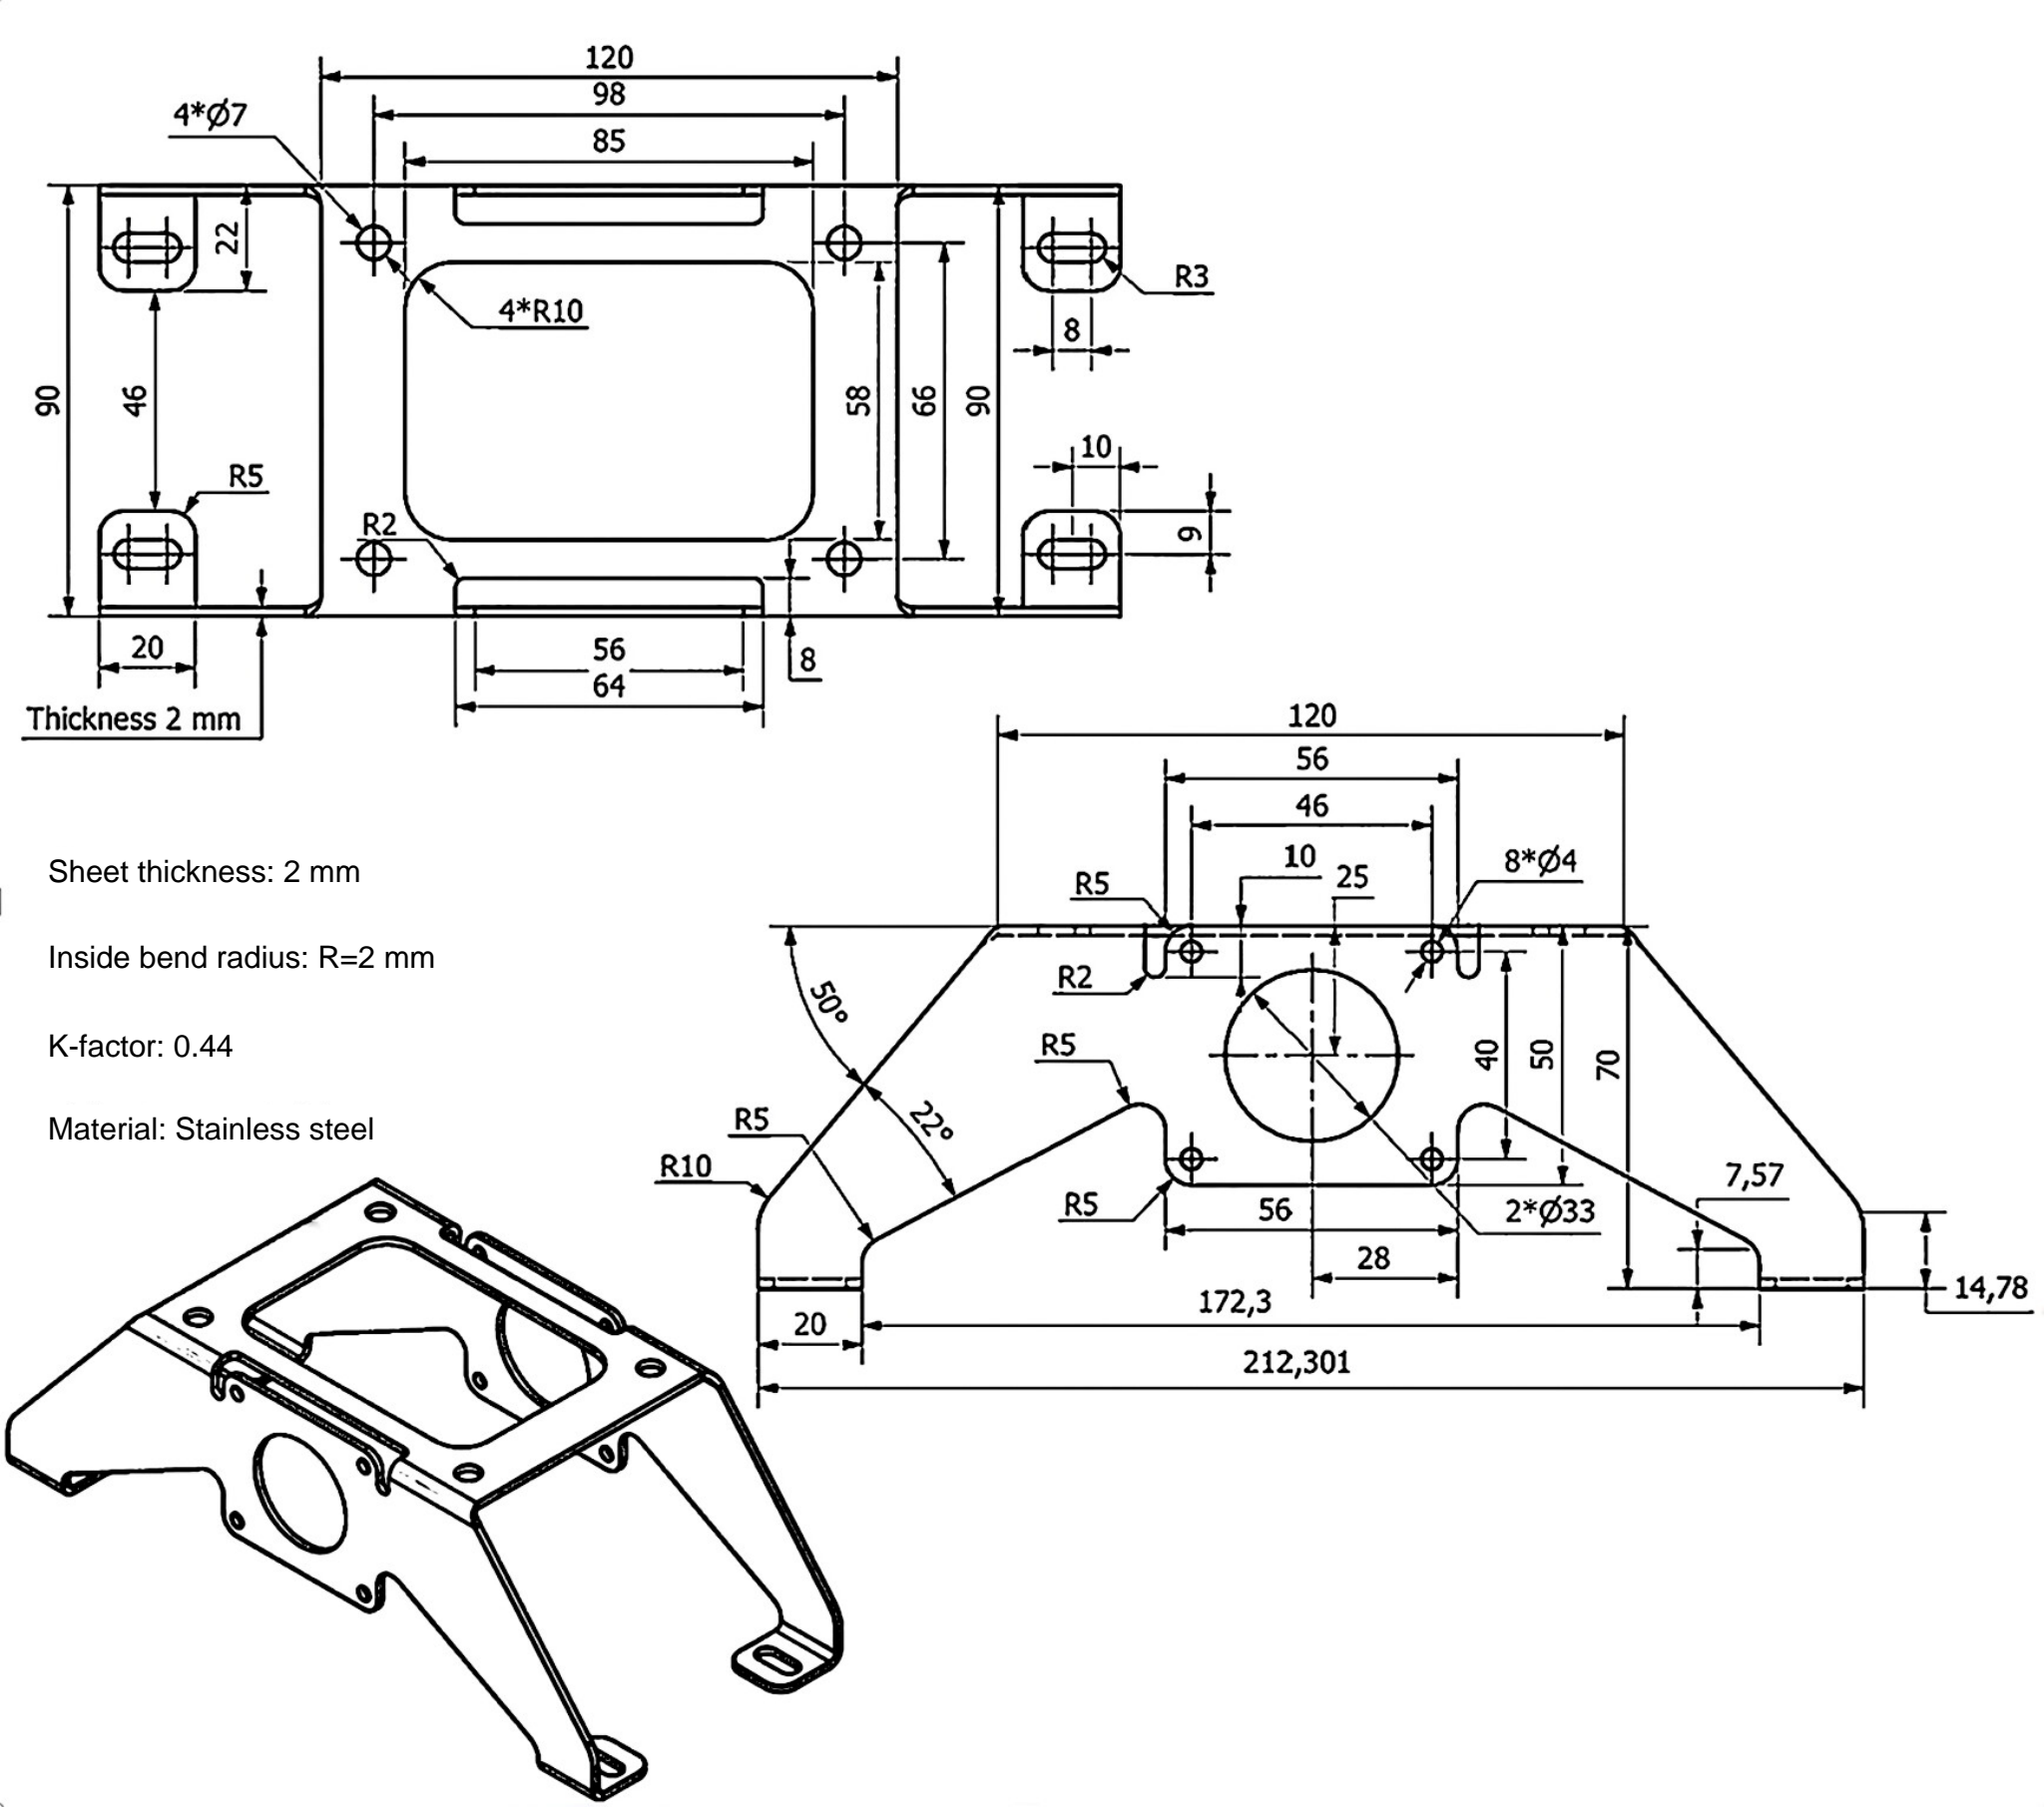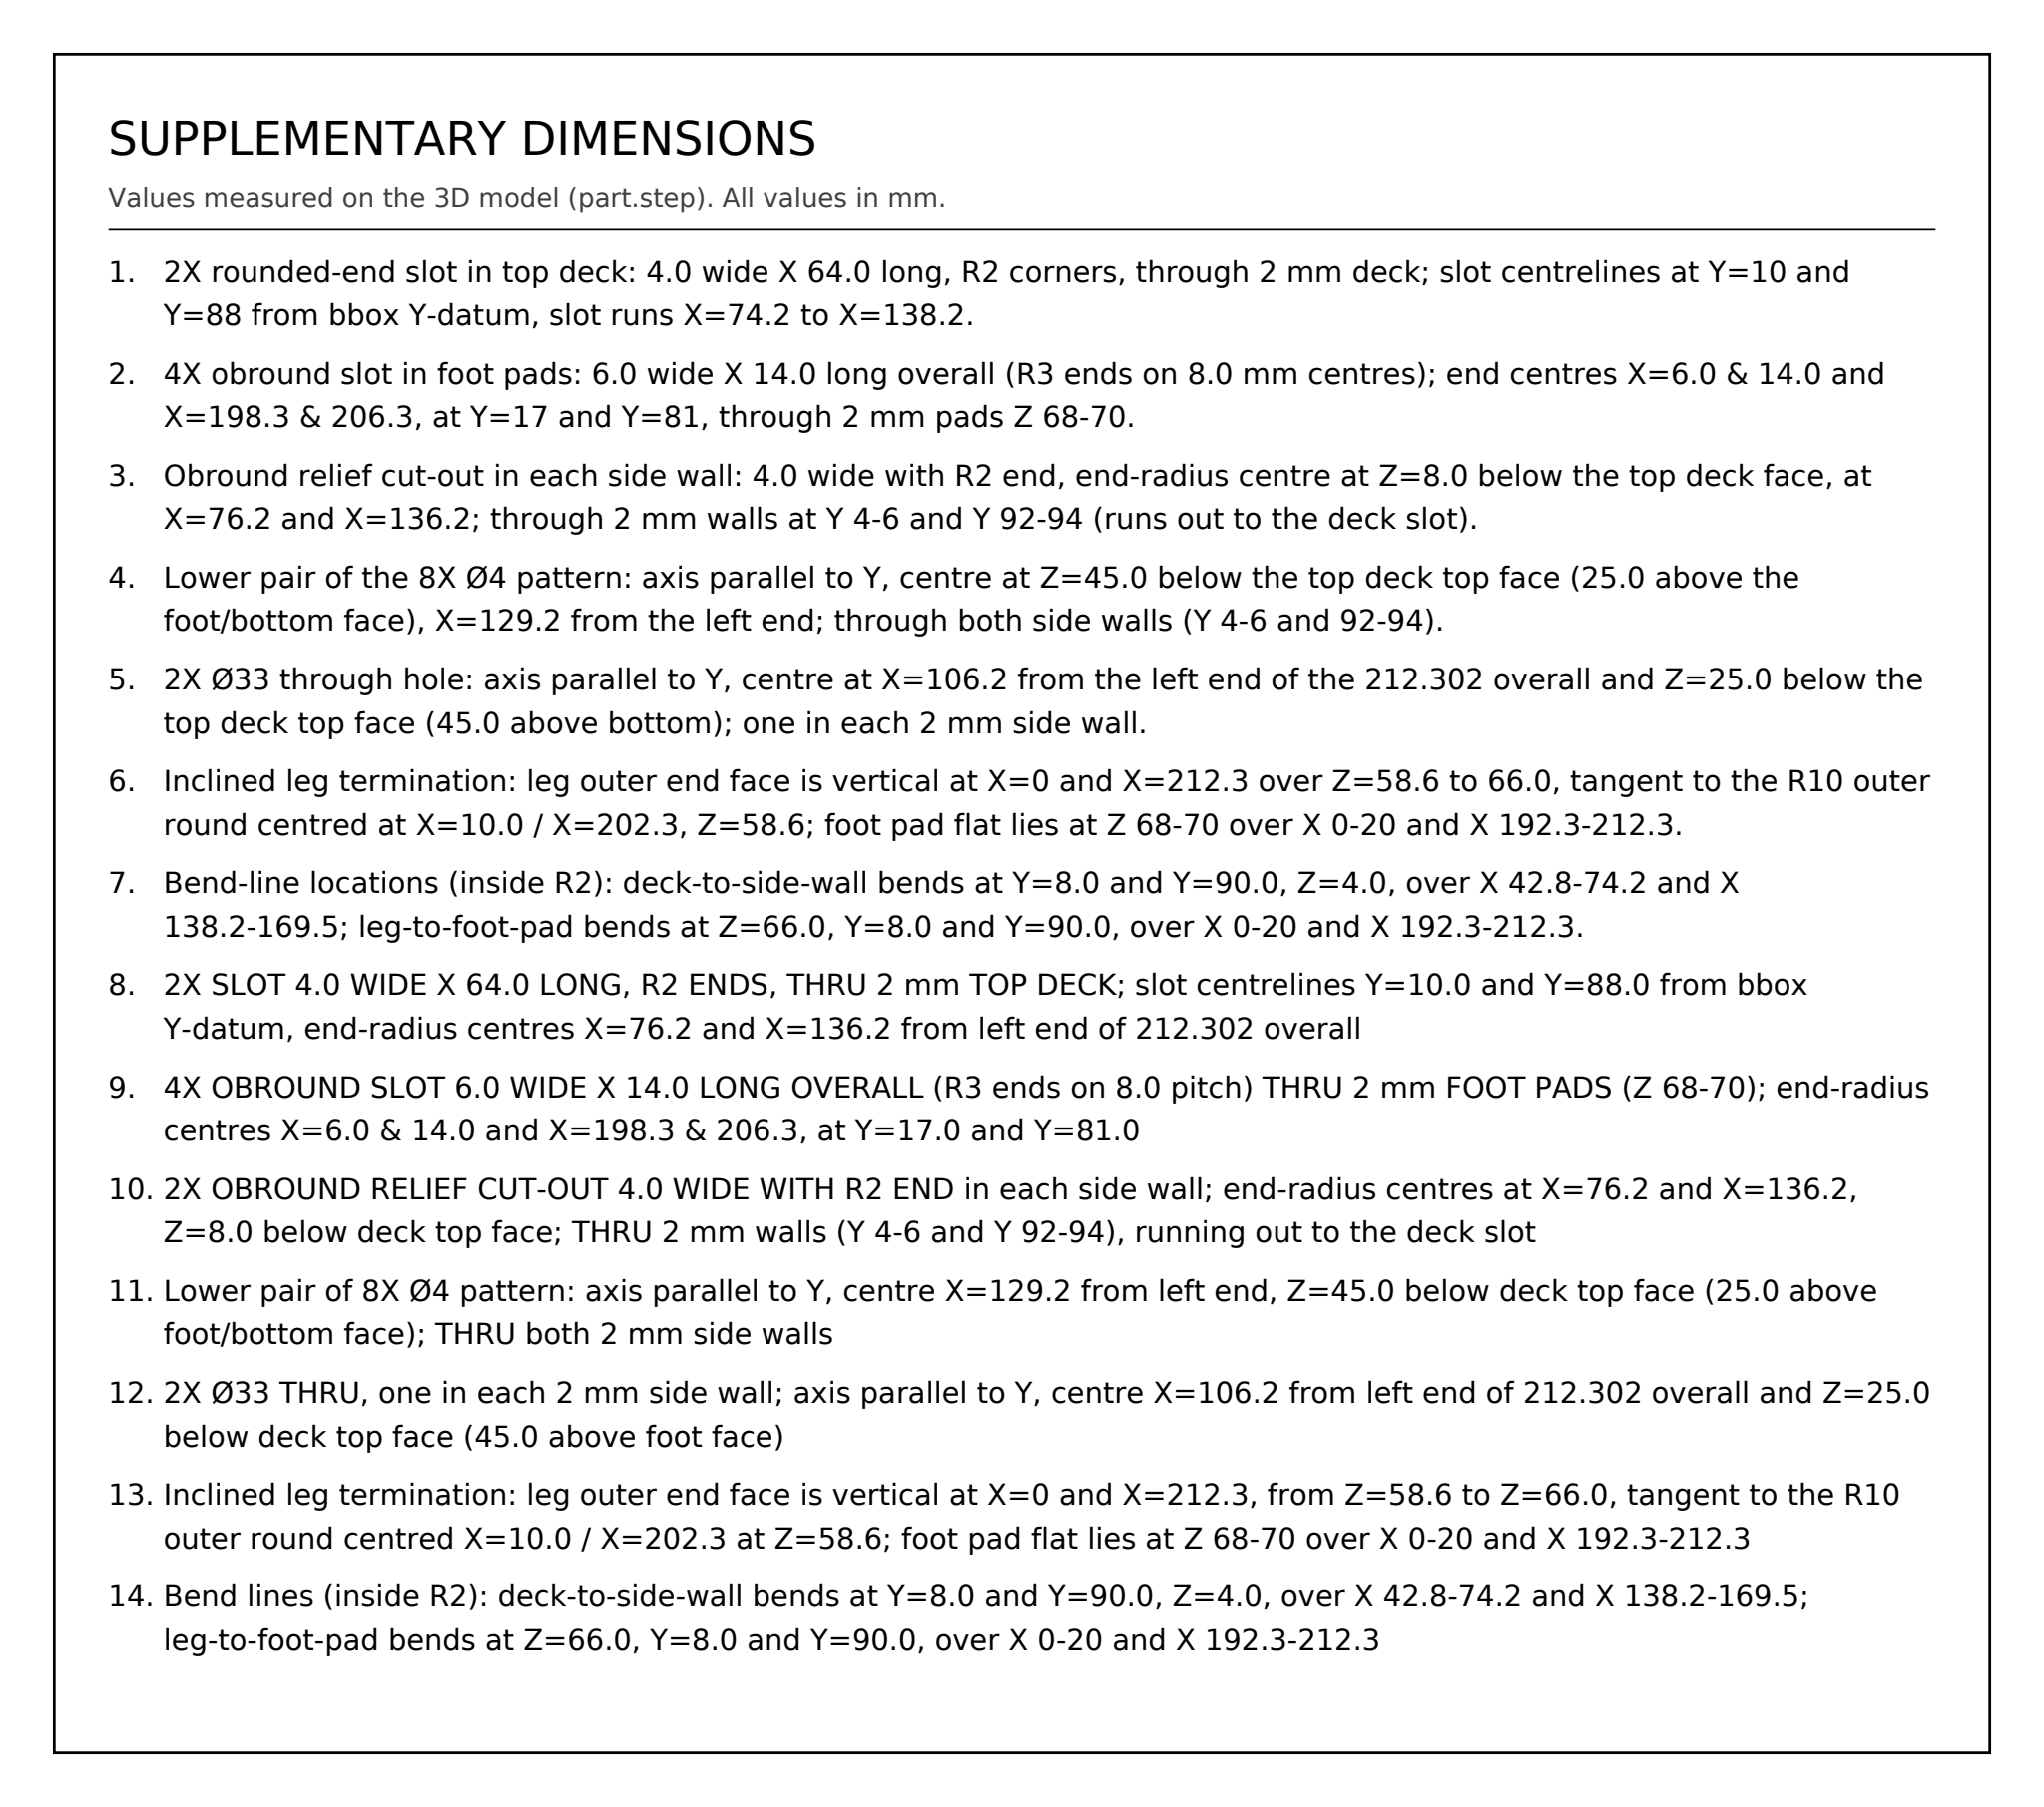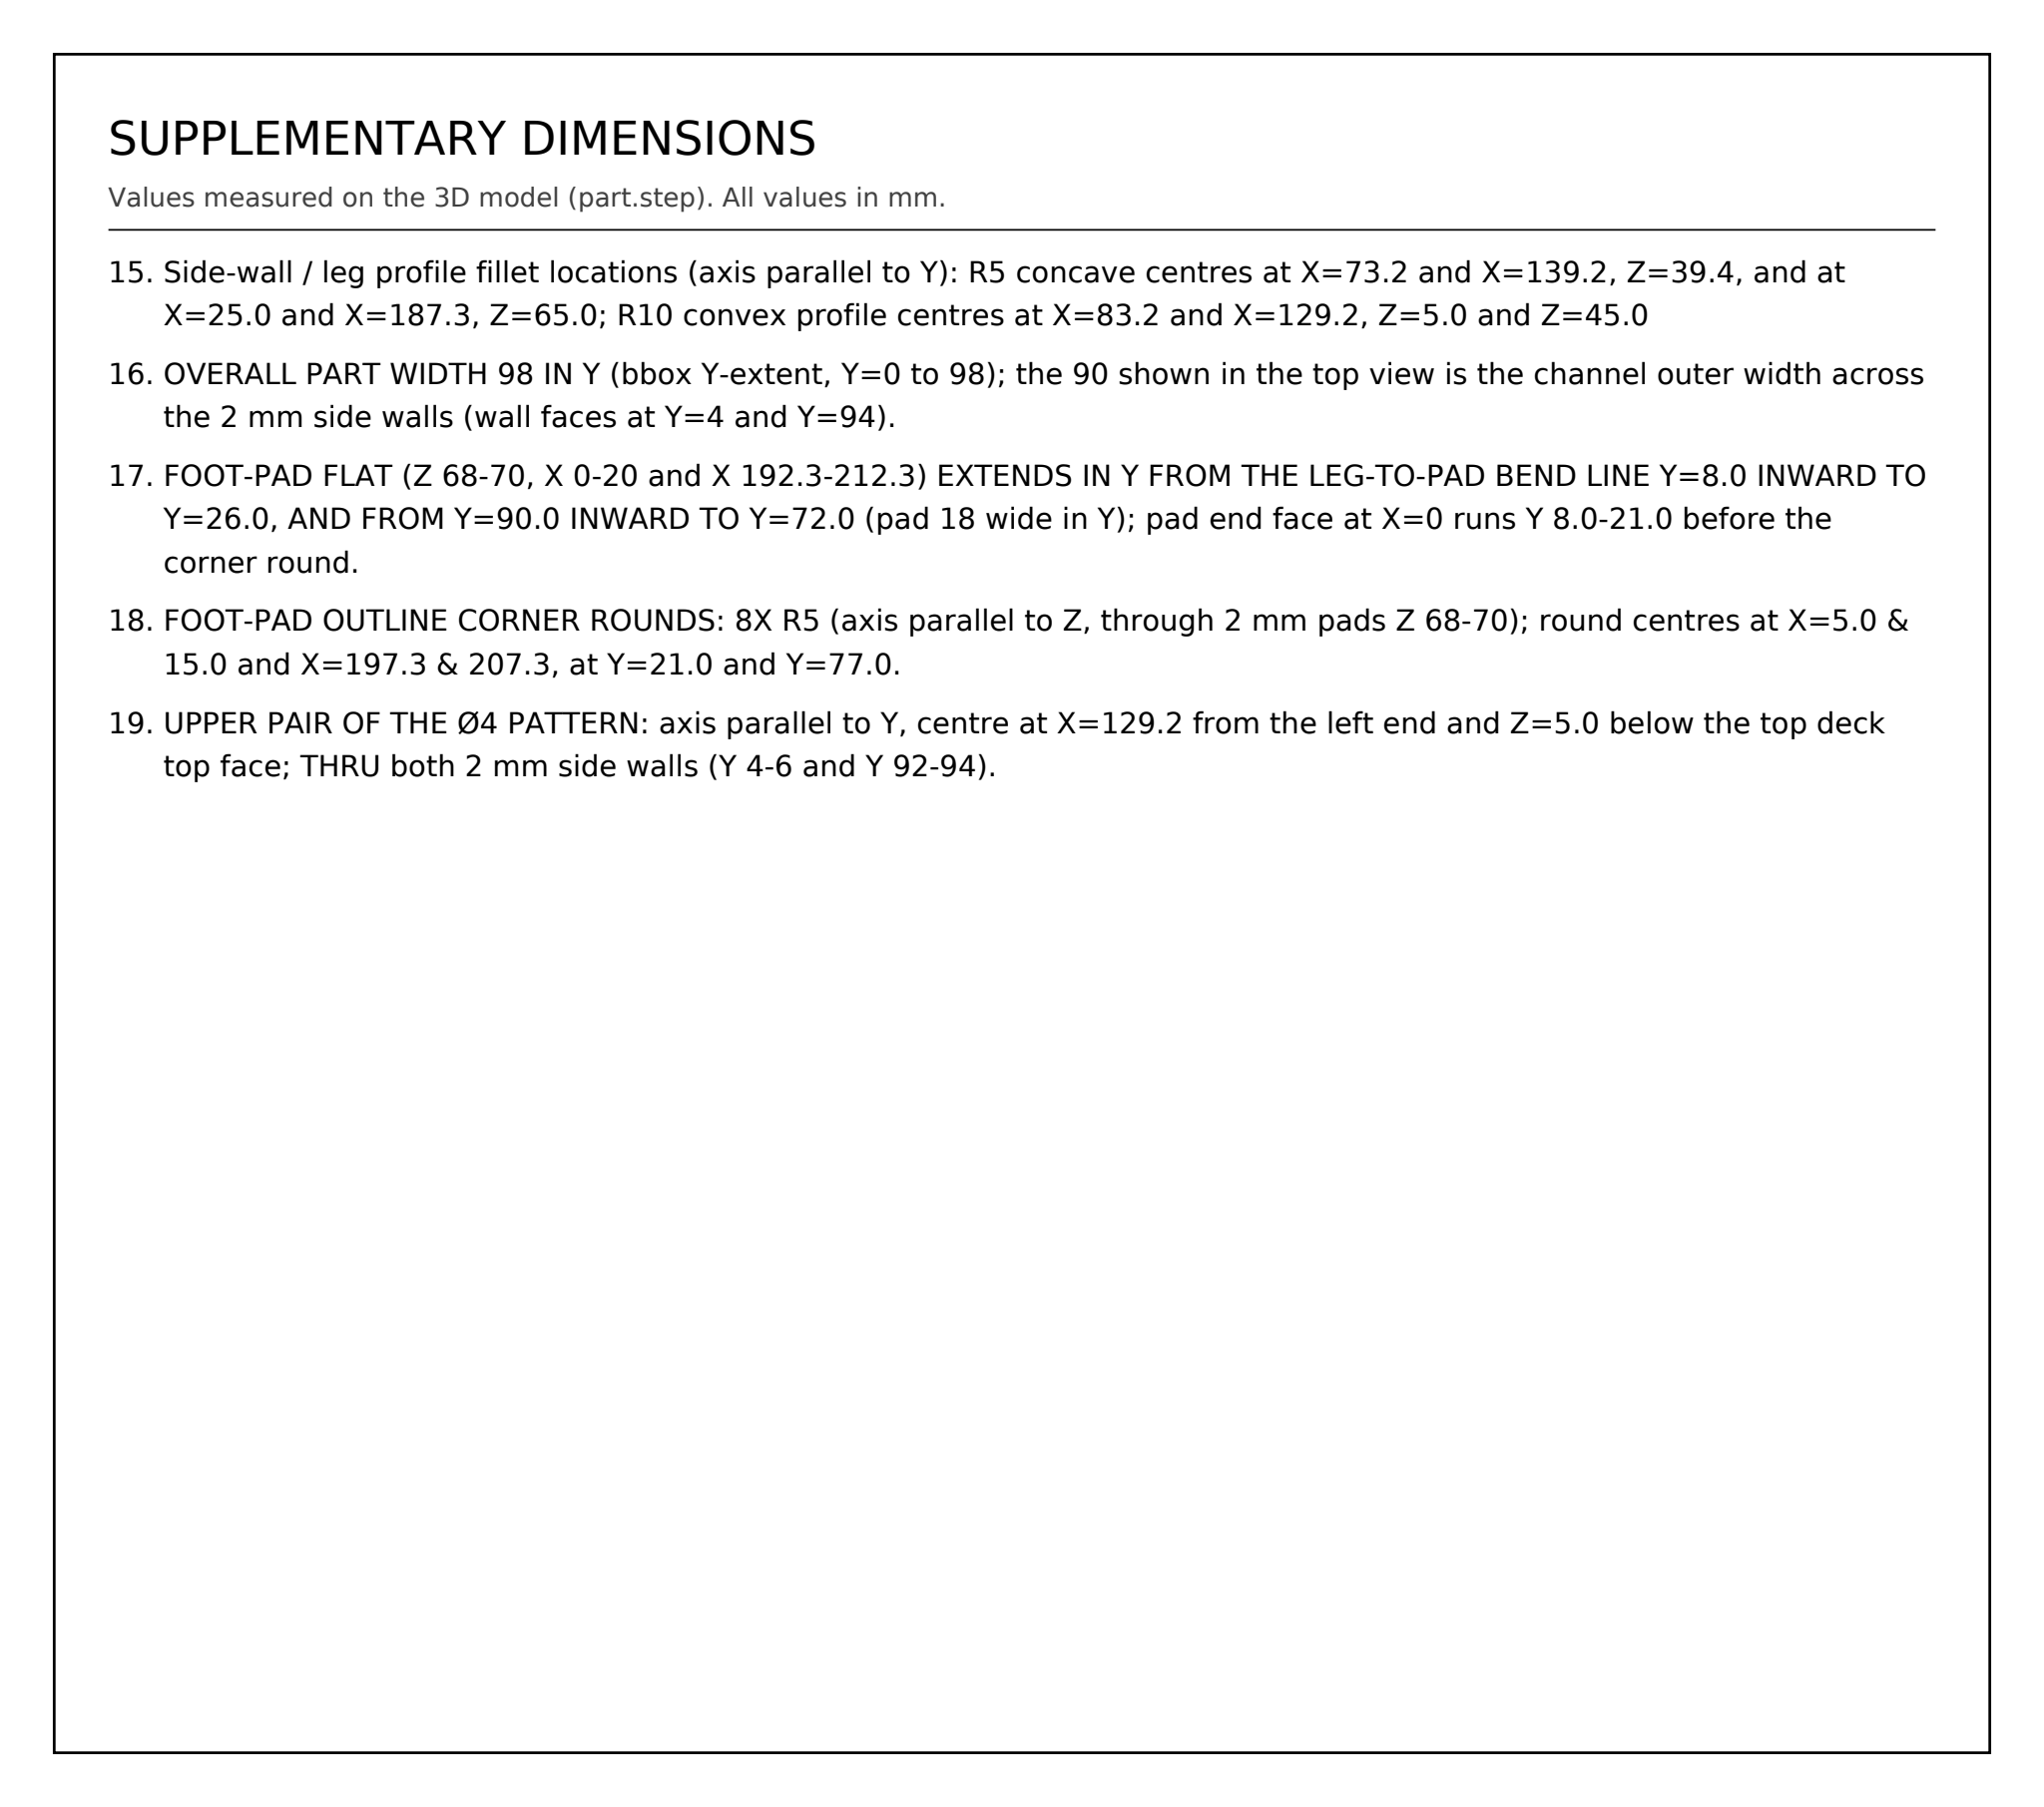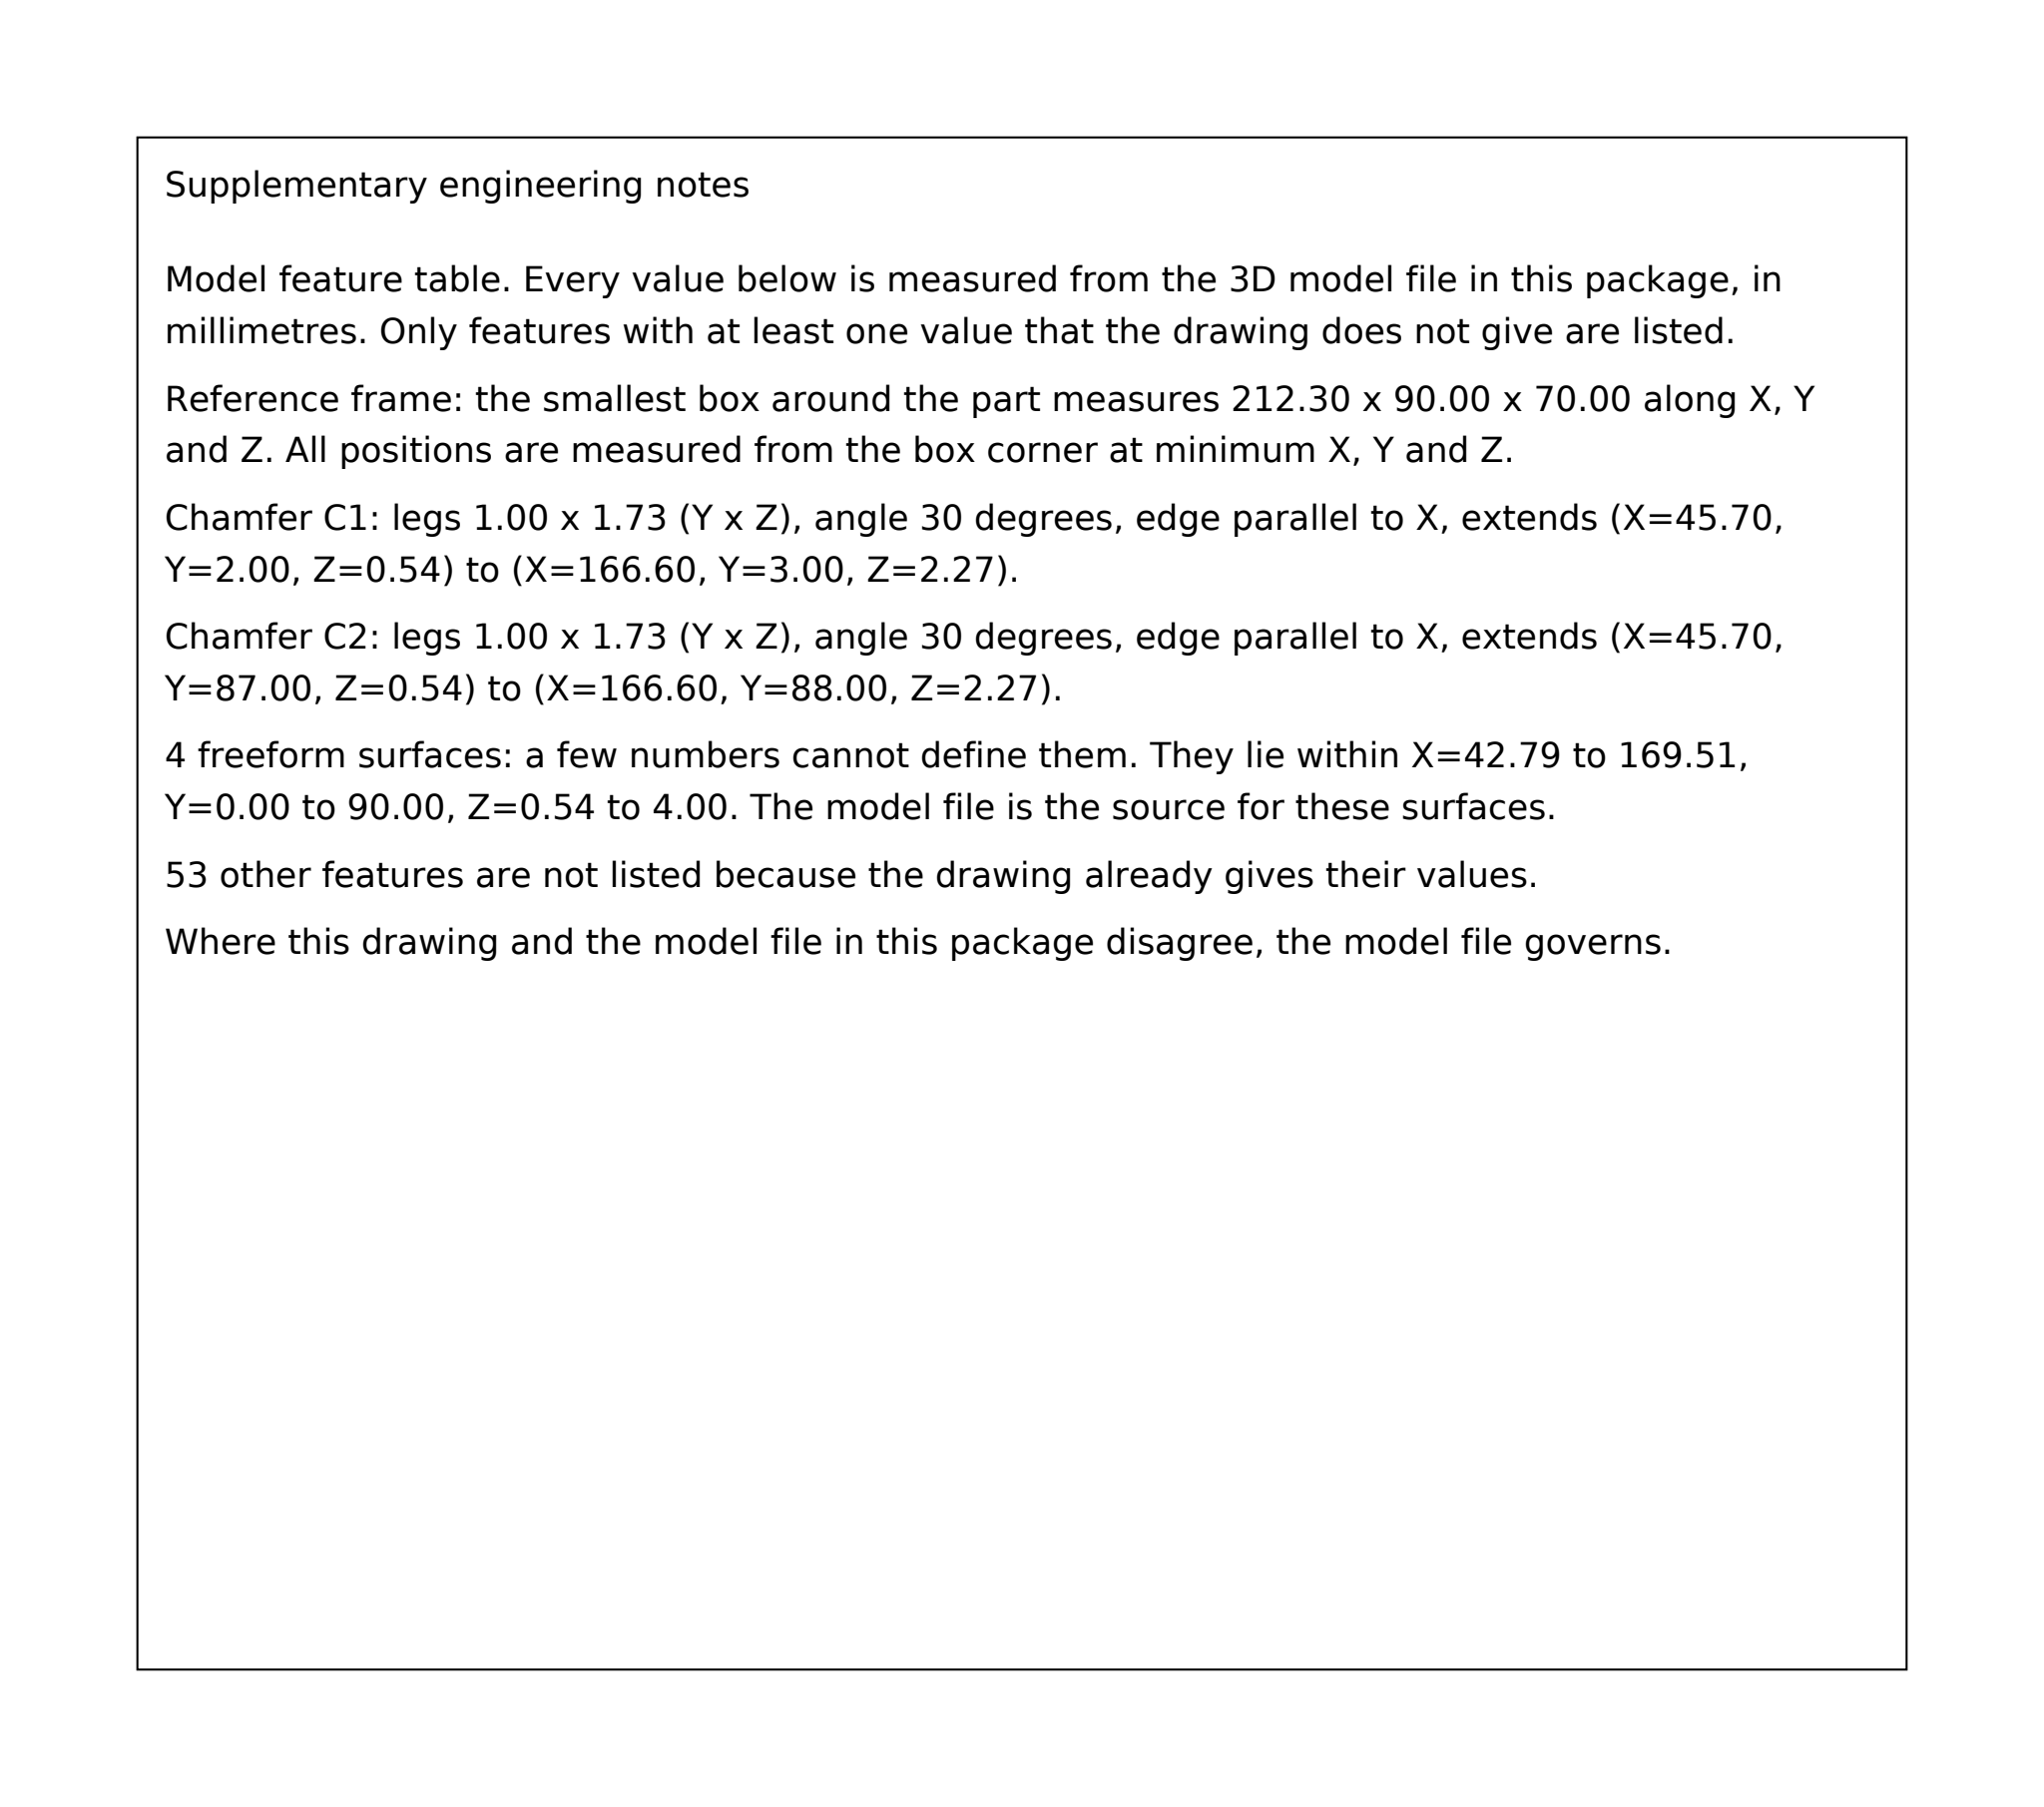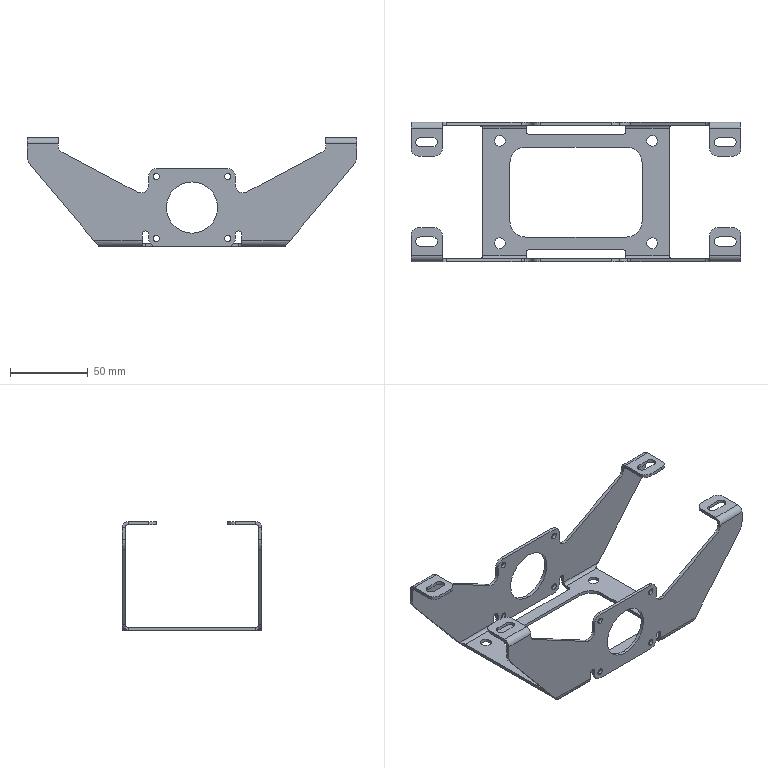Part | SolidWorks | mm | 1 solid | 202 faces | box 212.3 x 90 x 70 mm | volume 41125 mm3 | cylinder 100 | plane 98 | spline 4 | commonest cylinder face diameters 4 x34 10 x26 6 x12 7 x8 20 x8 8 x8 33 x4
Drawing notes:
2X rounded-end slot in top deck: 4.0 wide X 64.0 long, R2 corners, through 2 mm deck; slot centrelines at Y=10 and Y=88 from bbox Y-datum, slot runs X=74.2 to X=138.2. | from the solid: concave arc (R2) dia 4.0, z-axis, at (136.2,10),(76.2,10),(136.2,88),(76.2,88), from z 0.0 to 2.0
4X obround slot in foot pads: 6.0 wide X 14.0 long overall (R3 ends on 8.0 mm centres); end centres X=6.0 & 14.0 and X=198.3 & 206.3, at Y=17 and Y=81, through 2 mm pads Z 68-70. | from the solid: concave arc dia 6.0, z-axis, at (6,17),(14,17),(198.3,17),(206.3,17),(6,81),(14,81),(198.3,81),(206.3,81), from z 68.0 to 70.0
Obround relief cut-out in each side wall: 4.0 wide with R2 end, end-radius centre at Z=8.0 below the top deck face, at X=76.2 and X=136.2; through 2 mm walls at Y 4-6 and Y 92-94 (runs out to the deck slot). | from the solid: concave arc dia 4.0, y-axis, at (136.2, z=8.0) and (76.2, z=8.0), 180 deg, y 4.0-6.0 and 92.0-94.0
Lower pair of the 8X Ø4 pattern: axis parallel to Y, centre at Z=45.0 below the top deck top face (25.0 above the foot/bottom face), X=129.2 from the left end; through both side walls (Y 4-6 and 92-94). | from the solid: hole/bore dia 4.0, y-axis, at (129.2, z=45.0), from y 4.0 to 6.0 and y 92.0 to 94.0
2X Ø33 through hole: axis parallel to Y, centre at X=106.2 from the left end of the 212.302 overall and Z=25.0 below the top deck top face (45.0 above bottom); one in each 2 mm side wall. | from the solid: hole/bore dia 33.0, y-axis, at (106.2, z=25.0), from y 4.0 to 6.0 and y 92.0 to 94.0
Inclined leg termination: leg outer end face is vertical at X=0 and X=212.3 over Z=58.6 to 66.0, tangent to the R10 outer round centred at X=10.0 / X=202.3, Z=58.6; foot pad flat lies at Z 68-70 over X 0-20 and X 192.3-212.3. | from the solid: convex arc dia 20.0, y-axis, at (10, z=58.6) and (202.3, z=58.6), 40 deg; plane normal x at 0.0, extent y 4-6, z 58.6-66.0
Bend-line locations (inside R2): deck-to-side-wall bends at Y=8.0 and Y=90.0, Z=4.0, over X 42.8-74.2 and X 138.2-169.5; leg-to-foot-pad bends at Z=66.0, Y=8.0 and Y=90.0, over X 0-20 and X 192.3-212.3. | from the solid: concave arc dia 4.0, x-axis, at (y=8, z=4) and (y=90, z=4) from x 42.8-74.2 and 138.2-169.5; at (y=8, z=66) and (y=90, z=66) from x 0-20 and 192.3-212.3
2X SLOT 4.0 WIDE X 64.0 LONG, R2 ENDS, THRU 2 mm TOP DECK; slot centrelines Y=10.0 and Y=88.0 from bbox Y-datum, end-radius centres X=76.2 and X=136.2 from left end of 212.302 overall | from the solid: concave arc dia 4.0, axis z, at [76.2,10.0], [136.2,10.0], [76.2,88.0], [136.2,88.0], from z 0.0 to 2.0, 90 deg (deck slot corner radii)
4X OBROUND SLOT 6.0 WIDE X 14.0 LONG OVERALL (R3 ends on 8.0 pitch) THRU 2 mm FOOT PADS (Z 68-70); end-radius centres X=6.0 & 14.0 and X=198.3 & 206.3, at Y=17.0 and Y=81.0 | from the solid: concave arc dia 6.0, axis z, at [6.0,17.0],[14.0,17.0],[198.3,17.0],[206.3,17.0],[6.0,81.0],[14.0,81.0],[198.3,81.0],[206.3,81.0], from z 68.0 to 70.0, 180 deg
2X OBROUND RELIEF CUT-OUT 4.0 WIDE WITH R2 END in each side wall; end-radius centres at X=76.2 and X=136.2, Z=8.0 below deck top face; THRU 2 mm walls (Y 4-6 and Y 92-94), running out to the deck slot | from the solid: concave arc dia 4.0, axis y, at [76.2,null,8.0] and [136.2,null,8.0], from y 4.0 to 6.0 and y 92.0 to 94.0, 180 deg
Lower pair of 8X Ø4 pattern: axis parallel to Y, centre X=129.2 from left end, Z=45.0 below deck top face (25.0 above foot/bottom face); THRU both 2 mm side walls | from the solid: hole/bore dia 4.0, axis y, [129.2,null,45.0], from y 4.0 to 6.0 and y 92.0 to 94.0, 360 deg
2X Ø33 THRU, one in each 2 mm side wall; axis parallel to Y, centre X=106.2 from left end of 212.302 overall and Z=25.0 below deck top face (45.0 above foot face) | from the solid: hole/bore dia 33.0, axis y, [106.2,null,25.0], from y 4.0 to 6.0 and y 92.0 to 94.0, 360 deg
Inclined leg termination: leg outer end face is vertical at X=0 and X=212.3, from Z=58.6 to Z=66.0, tangent to the R10 outer round centred X=10.0 / X=202.3 at Z=58.6; foot pad flat lies at Z 68-70 over X 0-20 and X 192.3-212.3 | from the solid: axis_plane normal x at offset 0.0, extent y 4.0-6.0, z 58.6-66.0; convex arc dia 20.0, axis y, [10.0,null,58.6] and [202.3,null,58.6], 40 deg
Bend lines (inside R2): deck-to-side-wall bends at Y=8.0 and Y=90.0, Z=4.0, over X 42.8-74.2 and X 138.2-169.5; leg-to-foot-pad bends at Z=66.0, Y=8.0 and Y=90.0, over X 0-20 and X 192.3-212.3 | from the solid: concave arc dia 4.0, axis x, [null,8.0,4.0] and [null,90.0,4.0] from x 42.8-74.2 and 138.2-169.5; [null,8.0,66.0] and [null,90.0,66.0] from x 0-20 and 192.3-212.3
Side-wall / leg profile fillet locations (axis parallel to Y): R5 concave centres at X=73.2 and X=139.2, Z=39.4, and at X=25.0 and X=187.3, Z=65.0; R10 convex profile centres at X=83.2 and X=129.2, Z=5.0 and Z=45.0 | from the solid: concave arc dia 10.0, axis y, [73.2,null,39.4], [139.2,null,39.4], [25.0,null,65.0], [187.3,null,65.0]; convex arc dia 10.0, axis y, [83.2,null,5.0], [83.2,null,45.0], [129.2,null,5.0], [129.2,null,45.0]
OVERALL PART WIDTH 98 IN Y (bbox Y-extent, Y=0 to 98); the 90 shown in the top view is the channel outer width across the 2 mm side walls (wall faces at Y=4 and Y=94). | from the solid: bbox_xyz [212.302, 98.0, 70.0]; x=0 planes with extents y[4,6] and y[92,94] (side walls)
FOOT-PAD FLAT (Z 68-70, X 0-20 and X 192.3-212.3) EXTENDS IN Y FROM THE LEG-TO-PAD BEND LINE Y=8.0 INWARD TO Y=26.0, AND FROM Y=90.0 INWARD TO Y=72.0 (pad 18 wide in Y); pad end face at X=0 runs Y 8.0-21.0 before the corner round. | from the solid: axis_planes x=0 extent y[8,21] z[68,70] and y[77,90] z[68,70]; concave arcs dia 4 axis x at y=8/90, z=66 (leg-to-pad bends)
FOOT-PAD OUTLINE CORNER ROUNDS: 8X R5 (axis parallel to Z, through 2 mm pads Z 68-70); round centres at X=5.0 & 15.0 and X=197.3 & 207.3, at Y=21.0 and Y=77.0. | from the solid: convex arc (round/outer radius) dia 10.0 axis z at [5,21],[15,21],[197.3,21],[207.3,21],[5,77],[15,77],[197.3,77],[207.3,77], from z 68.0 to 70.0, 90 deg
UPPER PAIR OF THE Ø4 PATTERN: axis parallel to Y, centre at X=129.2 from the left end and Z=5.0 below the top deck top face; THRU both 2 mm side walls (Y 4-6 and Y 92-94). | from the solid: hole/bore dia 4.0 axis y at [129.2, null, 5.0], from y 4.0 to 6.0 and from y 92.0 to 94.0